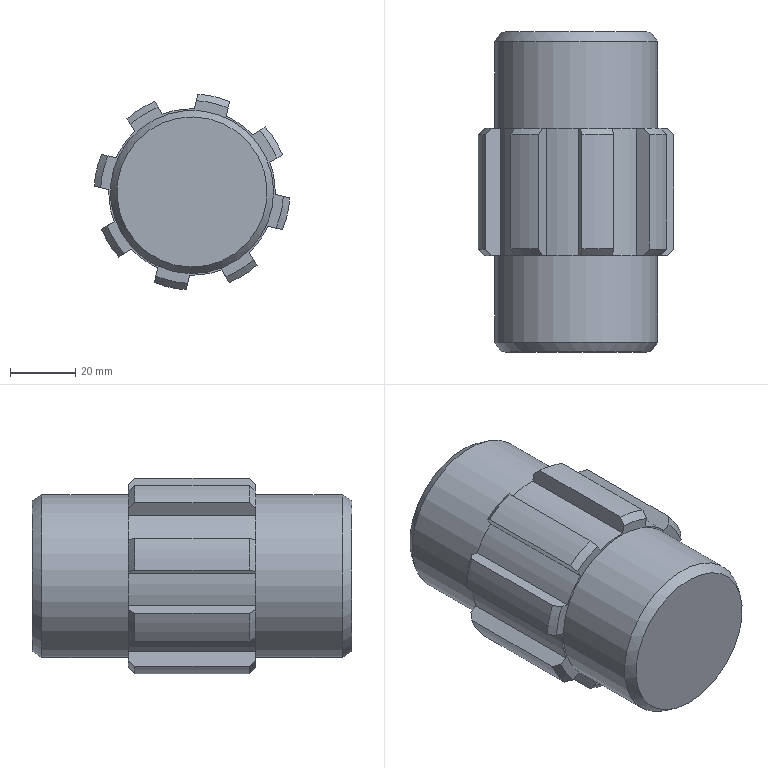Component | NX | MIDDLE_SHAFT_2 | 1 solid | 56 faces | volume 208395 mm3 | plane 20 | cylinder 18 | cone 18 | commonest cylinder face diameters 60 x8 51 x8 50 x2